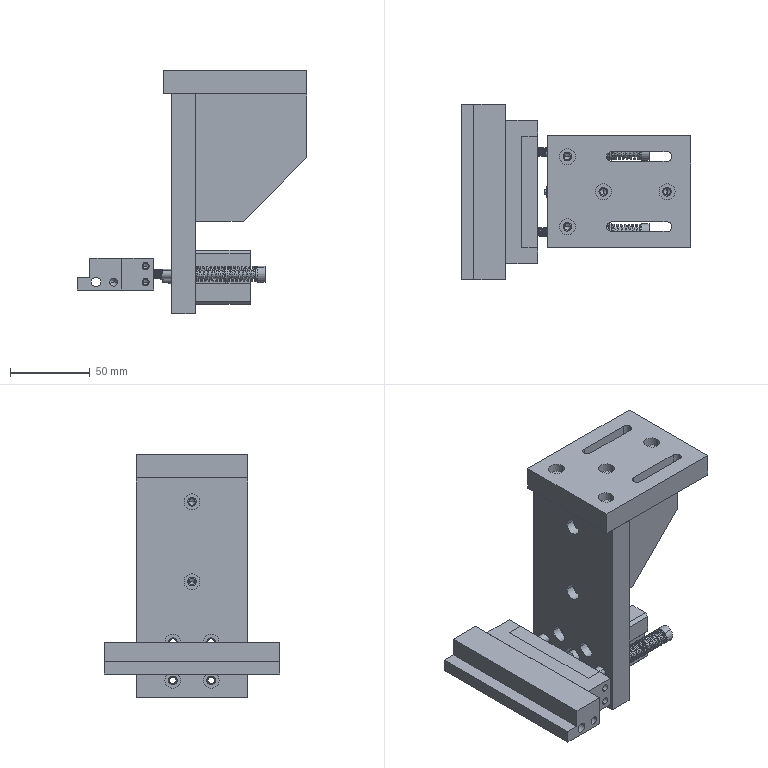Assembly | SolidWorks | mm | 17 component files | 17 solids | 584 faces | box 144.26 x 110 x 153 mm | volume 409165 mm3 | cylinder 278 | plane 182 | cone 92 | spline 30 | torus 2 | commonest cylinder face diameters 6 x82 10 x28 0.4 x26 5.5 x24 4.2 x20 4.134 x20 6.5 x16 3.3 x12
Bill of materials:
BeveledAluminumSupport | 1 |  | Solid prismatic block with a five-sided profile: a rectangle with one corner cut off at an angle. Two small holes in one narrow face.
EpoxyBoardSupportBlock | 1 |  | Rectangular bar with two round holes passing through the broad side face and two smaller holes in one end face.
hexagon socket head cap screws gb | 1 |  | Headed cylindrical pin or screw-like part: a short cylindrical head with a rounded edge and a smooth cylindrical shank with a chamfered tip.
OuterBagSealingBottomPlate | 1 |  | Flat rectangular plate with five round through holes and two parallel elongated slots.
OuterBagSealingCopperBlock | 1 |  | Long bar with an L-shaped (stepped) cross-section. One large hole runs lengthwise through it, the end face has a second hole, and a long face has two small holes.
OuterBagSealingGuideRod | 2 |  | Long slender headed screw: a cylindrical head, a long smooth shank, and a short threaded section at the tip.
OuterBagSealingSpring | 4 |  | Open helical coil of round-section wire with a constant outer diameter, roughly 8-9 turns, and an open center along the axis. The pitch looks even through the middle, the end turns sit closer together, and the end faces look flat. The shape matches a cylindrical helical compression-type spring.
OuterBagSealingSupportPlate | 1 |  | Thick rectangular plate with a pattern of holes through the broad face and two small holes in one narrow edge.
plain washers--product grade c gb | 2 |  | Flat annular ring with a plain washer shape.
SDA2015Axis | 1 |  | Headed pin: a large flat disc head and a cylindrical shank with a flat cut and a reduced step near the tip.
SDA2015Cylinder | 1 |  | Compact square body with an extruded profile: corners cut off at an angle, four corner through holes, a large central circular feature on the end face, slots along the sides, and a short cylindrical boss on one end.
U-shapedEpoxyBoard | 1 |  | Bracket bar with a C-shaped plan: a long web with a tab at each end sticking out to the same side. Each end tab has two holes, and the web has two holes.
Mates:
1. coincident | OuterBagSealingBottomPlate-1 face at (-17.085, 2.185, 71.225) dir (0, 0, -1) | BeveledAluminumSupport-1 face at (2.915, 44.685, 71.225) dir (0, 0, 1)
2. concentric | OuterBagSealingBottomPlate-1 face at (17.915, 37.185, 86.225) dir (0, 0, 1) r 5 | BeveledAluminumSupport-1 face at (17.915, 37.185, 71.225) dir (0, 0, 1) r 2.1
3. concentric | OuterBagSealingBottomPlate-1 face at (57.915, 37.185, 86.225) dir (0, 0, 1) r 2.75 | BeveledAluminumSupport-1 face at (57.915, 37.185, 71.225) dir (0, 0, 1) r 2.1
4. coincident | OuterBagSealingBottomPlate-1 face at (-17.085, 2.185, 71.225) dir (0, 0, -1) | OuterBagSealingSupportPlate-1 face at (-12.085, 2.185, 71.225) dir (0, 0, 1)
5. concentric | BeveledAluminumSupport-1 face at (2.915, 37.185, 56.225) dir (-1, 0, 0) r 2.1 | OuterBagSealingSupportPlate-1 face at (-12.085, 37.185, 56.225) dir (-1, 0, 0) r 2.75
6. coincident | BeveledAluminumSupport-1 face at (2.915, 44.685, 71.225) dir (-1, 0, 0) | OuterBagSealingSupportPlate-1 face at (2.915, 2.185, 71.225) dir (1, 0, 0)
7. concentric | EpoxyBoardSupportBlock-1 face at (-23.341, 62.185, -41.775) dir (1, 0, 0) r 3 | OuterBagSealingGuideRod-1 face at (41.659, 62.185, -41.775) dir (-1, 0, 0) r 3
8. concentric | EpoxyBoardSupportBlock-1 face at (-23.341, 12.185, -41.775) dir (1, 0, 0) r 3 | OuterBagSealingGuideRod-2 face at (41.659, 12.185, -41.775) dir (-1, 0, 0) r 3
9. coincident | EpoxyBoardSupportBlock-1 face at (-23.341, 2.185, -31.775) dir (0, -1, 0) | U-shapedEpoxyBoard-2 face at (-23.341, 2.185, -121.775) dir (0, 1, 0)
10. concentric | EpoxyBoardSupportBlock-1 face at (-28.341, 2.185, -36.775) dir (0, -1, 0) r 1.65 | U-shapedEpoxyBoard-2 face at (-28.341, -7.815, -36.775) dir (0, 1, 0) r 2.25
11. concentric | EpoxyBoardSupportBlock-1 face at (-28.341, 2.185, -46.775) dir (0, -1, 0) r 1.65 | U-shapedEpoxyBoard-2 face at (-28.341, -7.815, -46.775) dir (0, 1, 0) r 2.25
12. coincident | OuterBagSealingGuideRod-1 face at (46.659, 62.185, -41.775) dir (1, 0, 0) | OuterBagSealingGuideRod-2 face at (46.659, 12.185, -41.775) dir (1, 0, 0)
13. concentric | OuterBagSealingCopperBlock-1 face at (-43.341, 62.185, -41.775) dir (1, 0, 0) r 1.65 | U-shapedEpoxyBoard-2 edge at (-43.341, 62.185, -41.775) dir (1, 0, 0) r 2.25
14. concentric | OuterBagSealingCopperBlock-1 face at (-43.341, 12.185, -41.775) dir (1, 0, 0) r 1.65 | U-shapedEpoxyBoard-2 face at (-33.341, 12.185, -41.775) dir (1, 0, 0) r 2.25
15. coincident | OuterBagSealingCopperBlock-1 face at (-43.341, -17.815, -31.775) dir (1, 0, 0) | U-shapedEpoxyBoard-2 face at (-43.341, -7.815, -51.775) dir (-1, 0, 0)
16. coincident | EpoxyBoardSupportBlock-1 face at (-33.341, 72.185, -31.775) dir (-1, 0, 0) | OuterBagSealingGuideRod-2 face at (-33.341, 12.185, -41.775) dir (-1, 0, 0)
17. distance | OuterBagSealingSupportPlate-1 face at (-12.085, 2.185, -66.775) dir (0, 0, -1) | EpoxyBoardSupportBlock-1 face at (-23.341, 72.185, -51.775) dir (0, 0, -1)
18. distance | OuterBagSealingSupportPlate-1 face at (-12.085, 2.185, 71.225) dir (0, -1, 0) | U-shapedEpoxyBoard-2 face at (-33.341, -7.815, -41.775) dir (0, -1, 0)
19. coincident | OuterBagSealingSupportPlate-1 face at (2.915, 2.185, 71.225) dir (1, 0, 0) | Ultra-thinCylinderSDA2015-1/SDA2015Cylinder-1 face at (2.915, 20.185, -60.775) dir (-1, 0, 0)
20. concentric | OuterBagSealingSupportPlate-1 face at (-12.085, 37.185, -43.775) dir (1, 0, 0) r 6.5 | Ultra-thinCylinderSDA2015-1/SDA2015Axis-1 face at (12.415, 37.185, -43.775) dir (1, 0, 0) r 4
21. concentric | OuterBagSealingSupportPlate-1 face at (-12.085, 49.185, -55.775) dir (-1, 0, 0) r 2.75 | Ultra-thinCylinderSDA2015-1/SDA2015Cylinder-1 face at (7.848, 49.185, -55.775) dir (1, 0, 0) r 2.067
22. concentric | Ultra-thinCylinderSDA2015-1/SDA2015Axis-1 face at (12.415, 37.185, -43.775) dir (1, 0, 0) r 4 | hexagon socket head cap screws gb-1 face at (-11.585, 37.185, -43.775) dir (-1, 0, 0) r 0.8
23. coincident | Ultra-thinCylinderSDA2015-1/SDA2015Axis-1 face at (-17.585, 34.113, -47.512) dir (-1, 0, 0) | hexagon socket head cap screws gb-1 face at (-17.585, 37.185, -43.775) dir (1, 0, 0)
24. concentric | OuterBagSealingGuideRod-2 face at (-33.341, 12.185, -41.775) dir (1, 0, 0) r 5 | OuterBagSealingSpring-1 axis at (124.141, 12.185, -41.775) dir (-1, 0, 0)
25. coincident | OuterBagSealingGuideRod-2 face at (41.659, 12.185, -41.775) dir (-1, 0, 0) | OuterBagSealingSpring-1 face at (41.659, 17.407, -20.061) dir (1, 0, 0)
26. concentric | OuterBagSealingGuideRod-2 face at (41.659, 12.185, -41.775) dir (-1, 0, 0) r 3 | plain washers--product grade c gb-2 face at (22.088, 12.185, -41.775) dir (1, 0, 0) r 2.75
27. coincident | OuterBagSealingSpring-1 face at (23.088, 17.407, -20.061) dir (-1, 0, 0) | plain washers--product grade c gb-2 face at (23.088, 12.185, -41.775) dir (1, 0, 0)
28. concentric | OuterBagSealingGuideRod-2 face at (41.659, 12.185, -41.775) dir (-1, 0, 0) r 3 | OuterBagSealingSpring-2 axis at (104.57, 12.185, -41.775) dir (-1, 0, 0)
29. coincident | plain washers--product grade c gb-2 face at (22.088, 12.185, -41.775) dir (-1, 0, 0) | OuterBagSealingSpring-2 face at (22.088, 17.407, -20.061) dir (1, 0, 0)
30. concentric | OuterBagSealingGuideRod-1 face at (41.659, 62.185, -41.775) dir (-1, 0, 0) r 3 | OuterBagSealingSpring-3 axis at (124.141, 62.185, -41.775) dir (-1, 0, 0)
31. concentric | OuterBagSealingGuideRod-1 face at (41.659, 62.185, -41.775) dir (-1, 0, 0) r 3 | OuterBagSealingSpring-4 axis at (104.57, 62.185, -41.775) dir (-1, 0, 0)
32. concentric | OuterBagSealingGuideRod-1 face at (41.659, 62.185, -41.775) dir (-1, 0, 0) r 3 | plain washers--product grade c gb-3 face at (22.088, 62.185, -41.775) dir (1, 0, 0) r 2.75
33. coincident | OuterBagSealingGuideRod-1 face at (41.659, 62.185, -41.775) dir (-1, 0, 0) | OuterBagSealingSpring-3 face at (41.659, 67.407, -20.061) dir (1, 0, 0)
34. coincident | plain washers--product grade c gb-3 face at (23.088, 62.185, -41.775) dir (1, 0, 0) | OuterBagSealingSpring-3 face at (23.088, 67.407, -20.061) dir (-1, 0, 0)
35. coincident | plain washers--product grade c gb-3 face at (22.088, 62.185, -41.775) dir (-1, 0, 0) | OuterBagSealingSpring-4 face at (22.088, 76.144, -59.208) dir (1, 0, 0)
36. concentric | SDA2015Cylinder-1 face at (3.166, 22.961, 20.042) dir (1, 0, 0) r 4 | SDA2015Axis-1 face at (14.166, 22.961, 20.042) dir (1, 0, 0) r 4